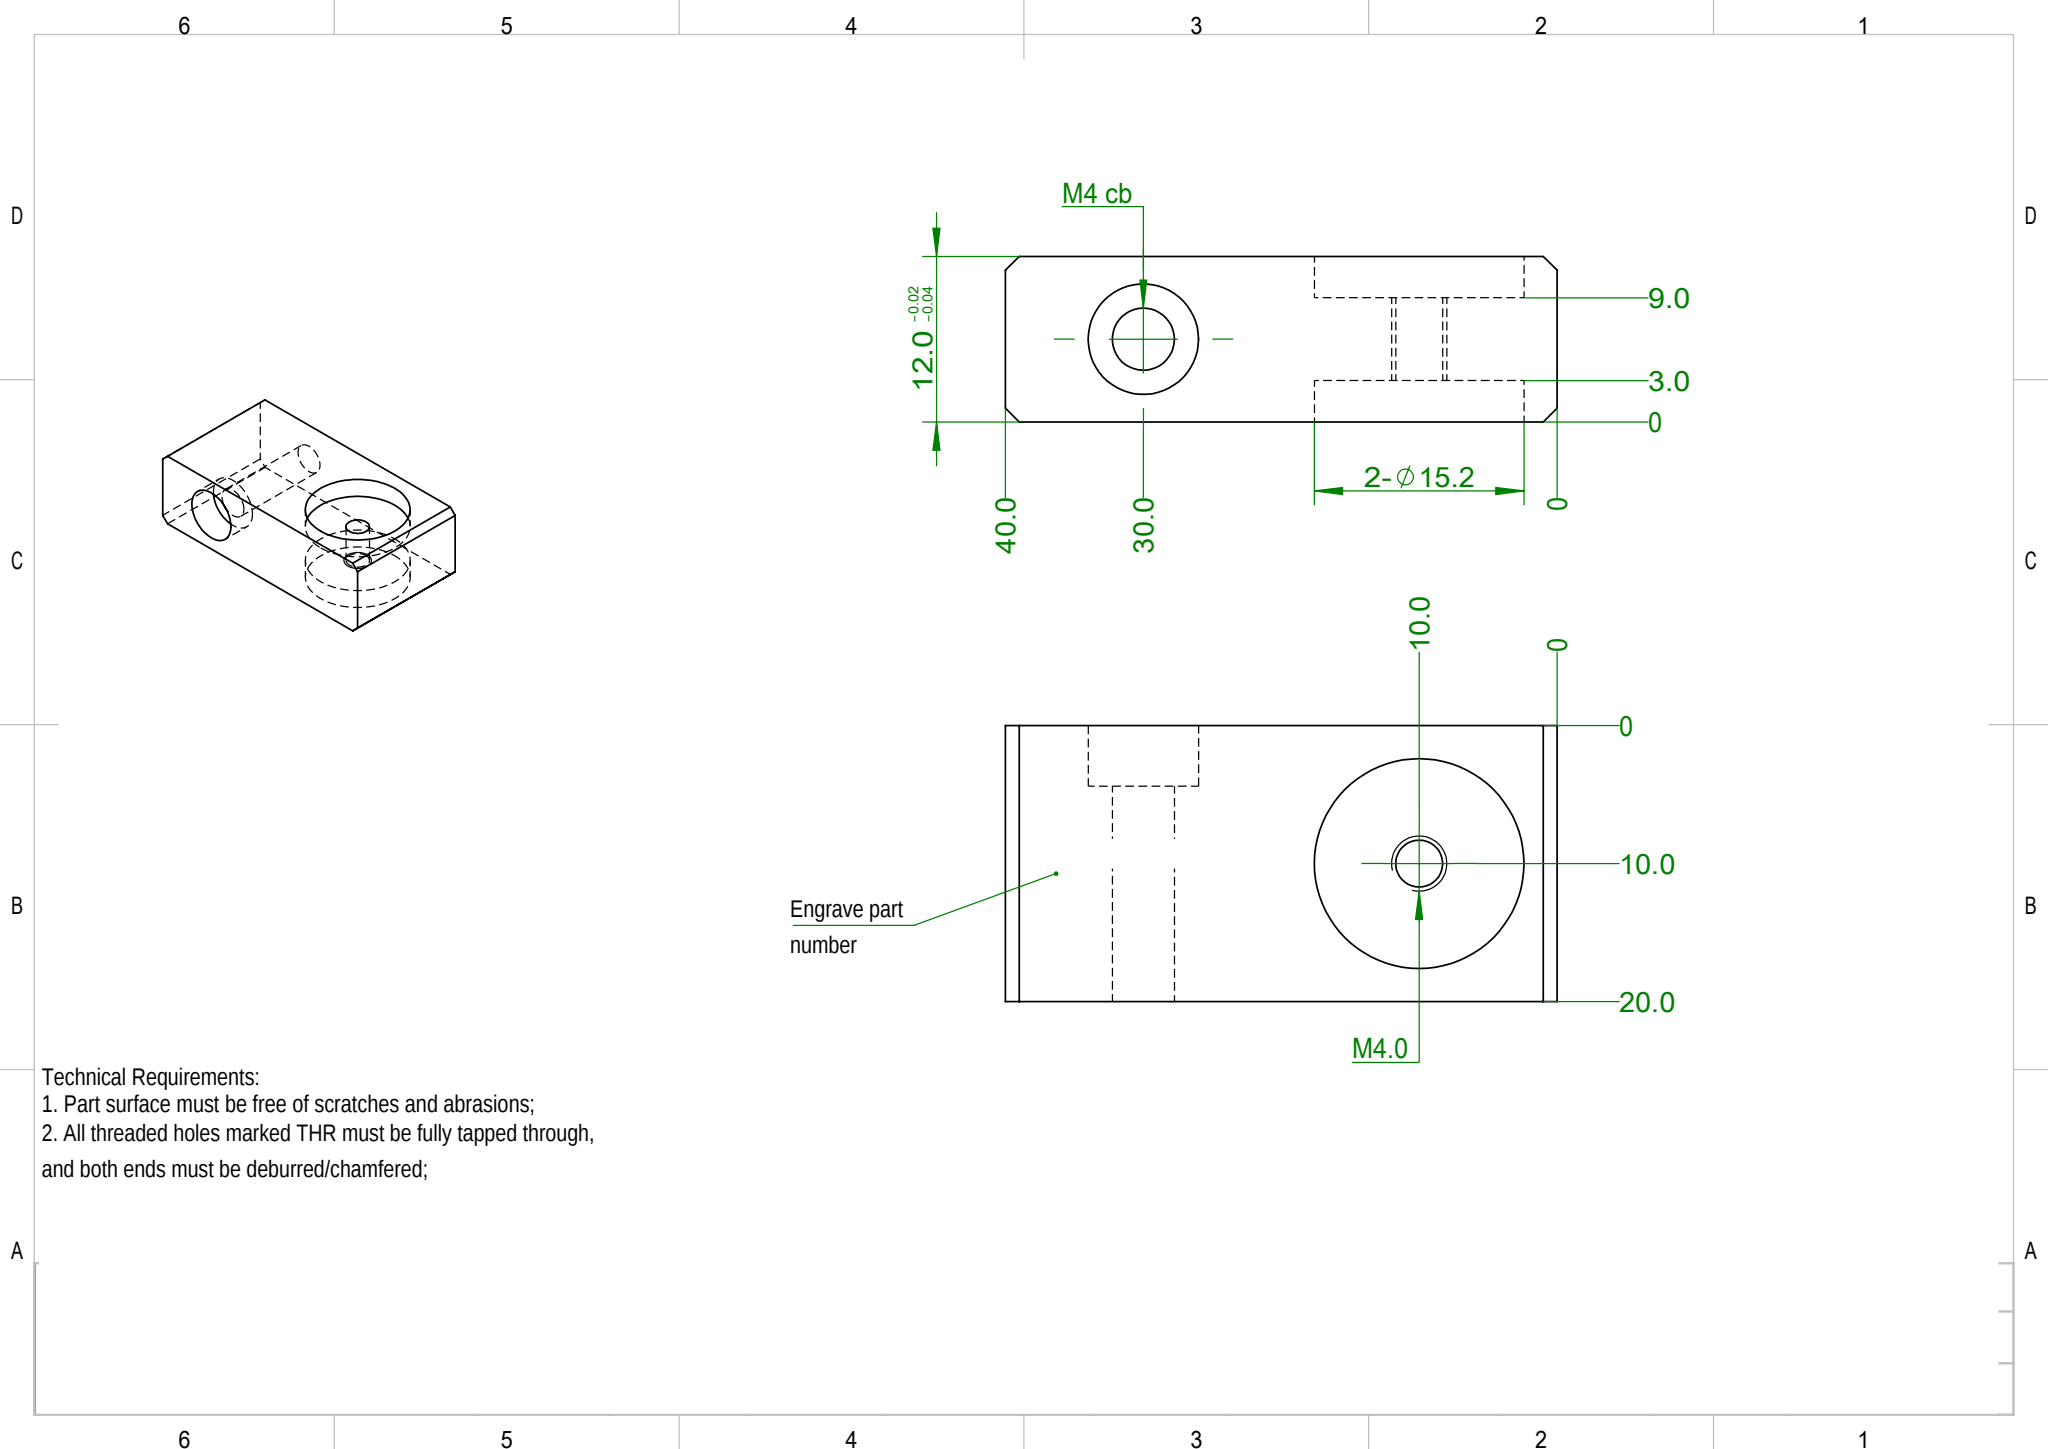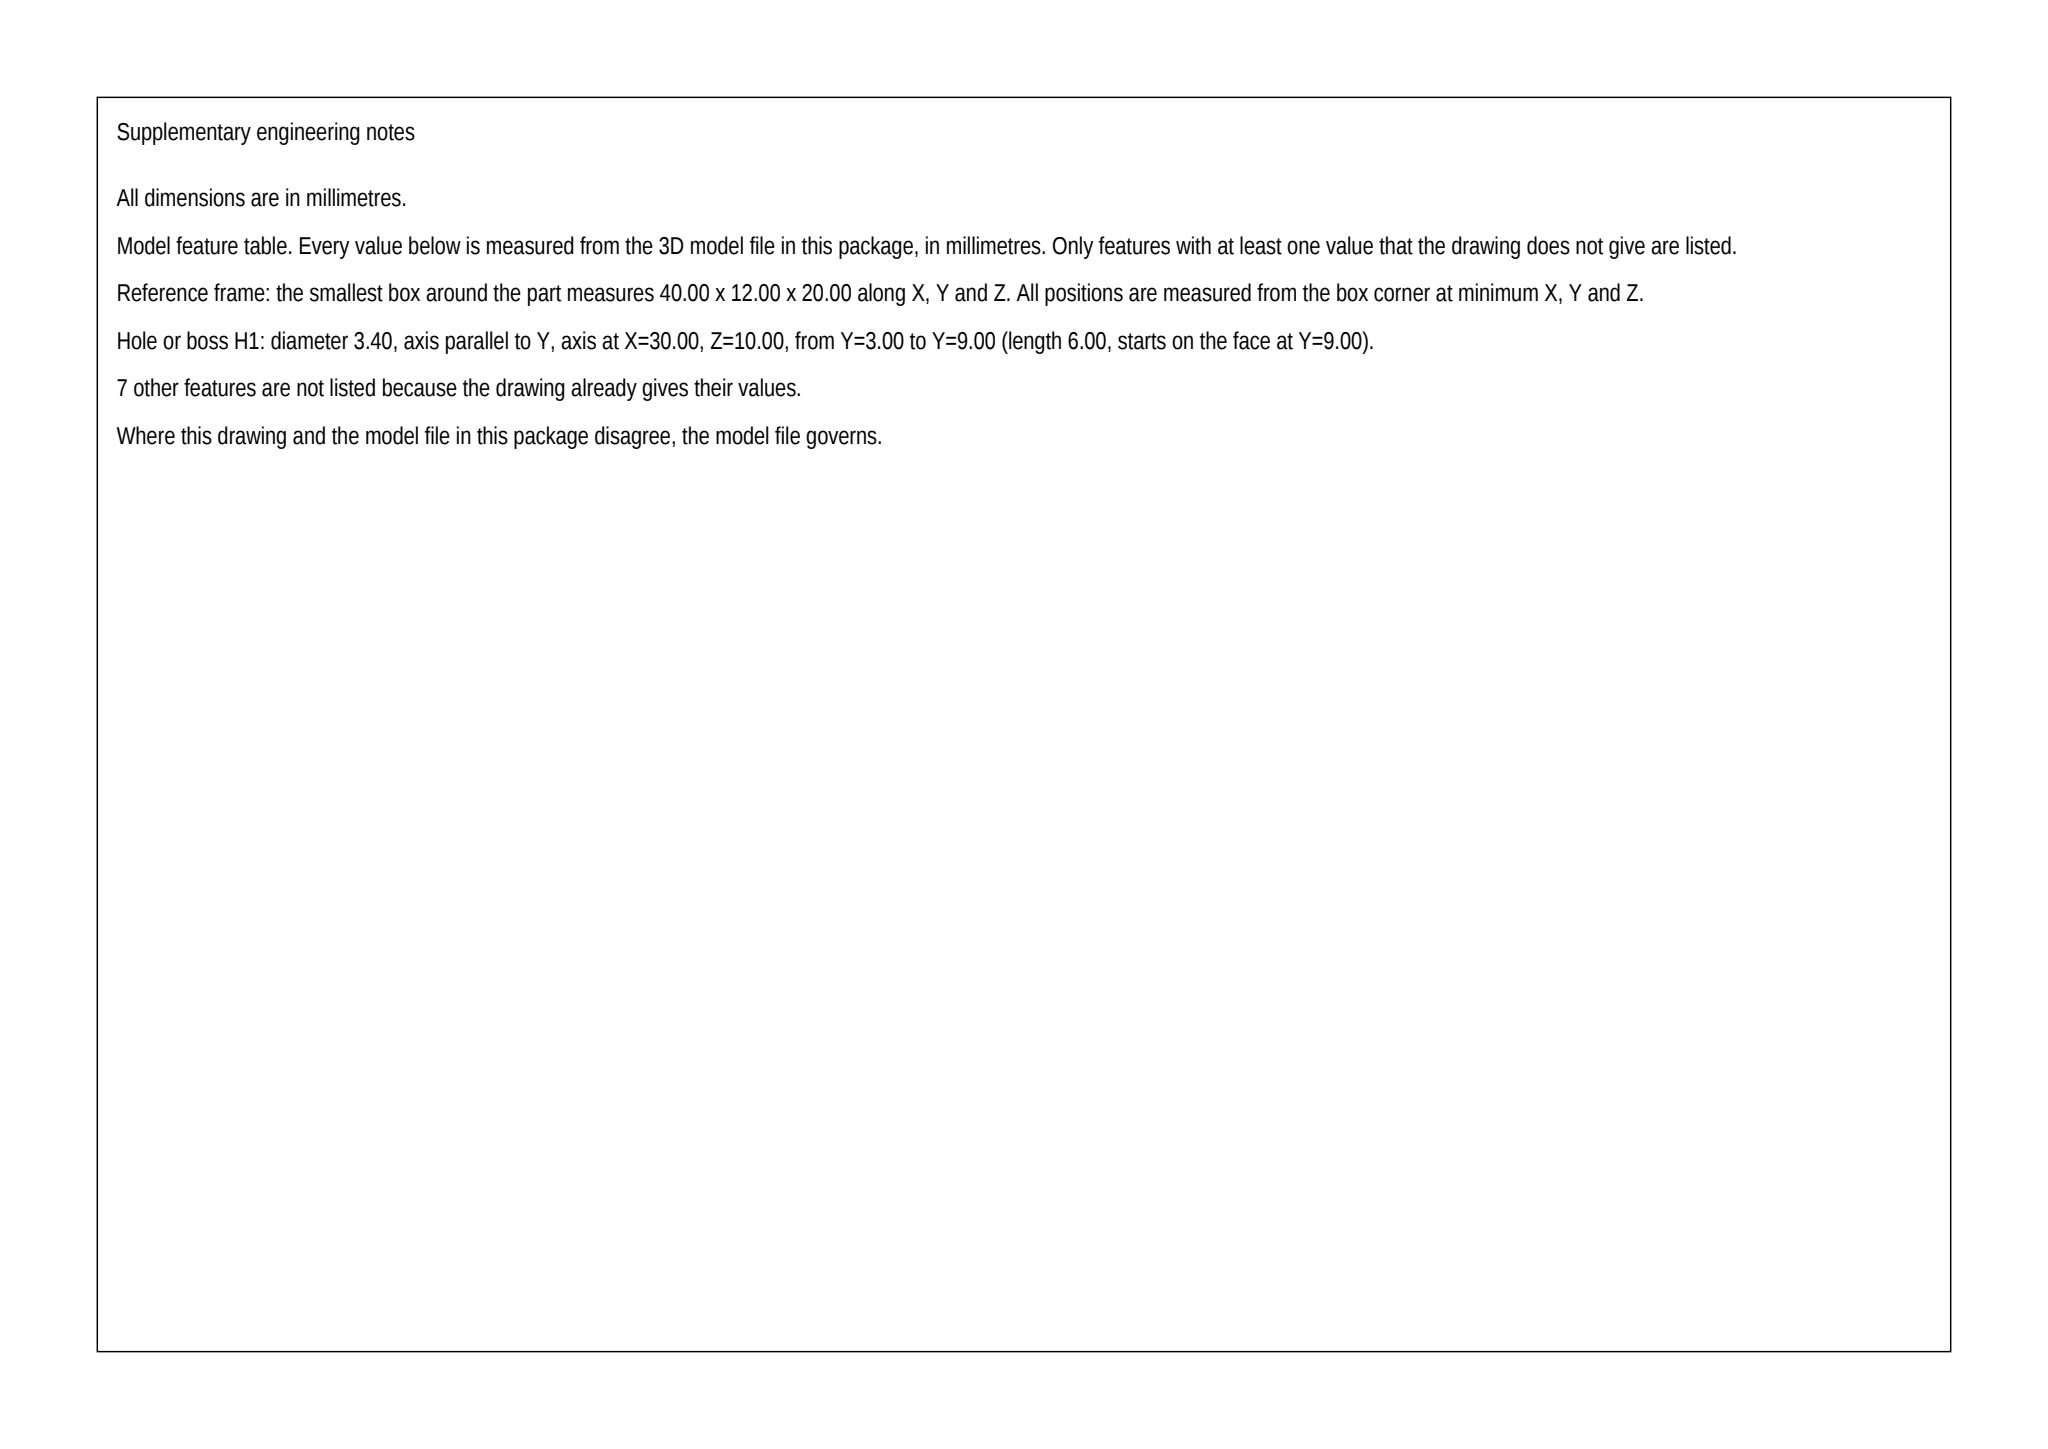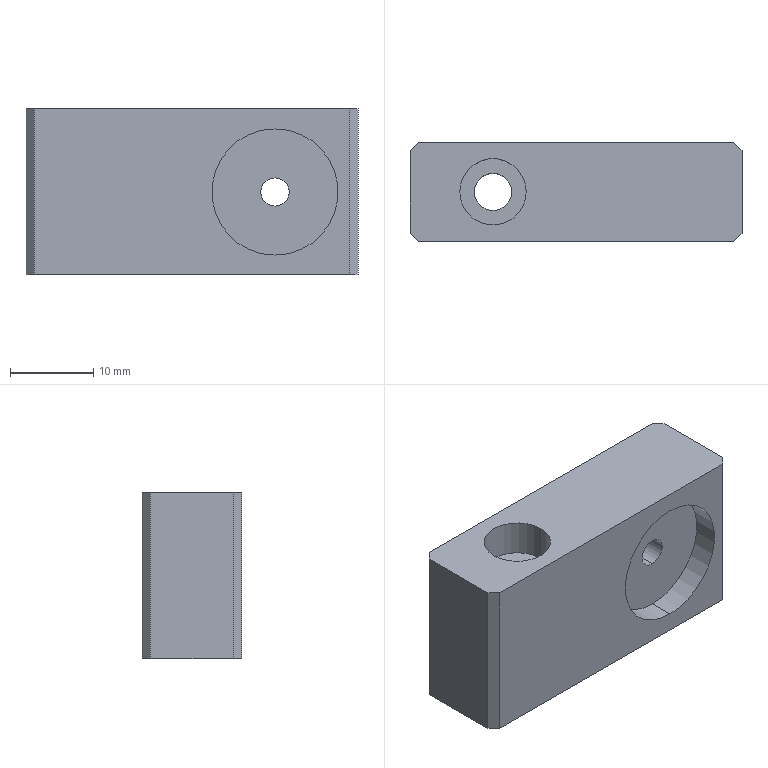Part | SolidWorks | mm | 1 solid | 23 faces | box 40 x 12 x 20 mm | volume 7947 mm3 | plane 13 | cylinder 10 | commonest cylinder face diameters 15.2 x4 8 x2 4.5 x2 3.4 x2
build123d program:
from build123d import *

# Parameters (mm, degrees)
SKETCH1_W                                       = 20
SKETCH1_H                                       = 12
BOSS_EXTRUDE1_DEPTH                             = 20
SKETCH4_R                                       = 7.6
CUT_EXTRUDE1_DEPTH                              = 3
SKETCH5_R                                       = 1.7
CUT_EXTRUDE2_DEPTH                              = 10
MOVE_FACE1_BY                                   = 20
M4_HEX_SOCKET_HEAD_CAP_SCREW_CBORE1_D           = 4.5
M4_HEX_SOCKET_HEAD_CAP_SCREW_CBORE1_CBORE_D     = 8
M4_HEX_SOCKET_HEAD_CAP_SCREW_CBORE1_CBORE_DEPTH = 4.4
CUT_EXTRUDE3_START                              = -3
SKETCH9_R                                       = 7.6
CUT_EXTRUDE3_DEPTH                              = 3
CHAMFER1_SIZE                                   = 1


with BuildPart() as part:
    # Sketch1 → Boss-Extrude1 (new body)
    with BuildSketch(Plane.XY):
        Rectangle(SKETCH1_W, SKETCH1_H)
    extrude(amount=BOSS_EXTRUDE1_DEPTH)

    # Sketch4 → Cut-Extrude1 (cut)
    with BuildSketch(Plane.XZ.offset(6)):
        with Locations(Location((0, 10, 0), (0, 0, 270))):
            Circle(SKETCH4_R)
    extrude(amount=-CUT_EXTRUDE1_DEPTH, mode=Mode.SUBTRACT)

    # Sketch5 → Cut-Extrude2 (cut)
    with BuildSketch(Plane.XZ.offset(3)):
        with Locations(Location((0, 10, 0), (0, 0, 270))):
            Circle(SKETCH5_R)
    extrude(amount=-CUT_EXTRUDE2_DEPTH, mode=Mode.SUBTRACT)

    # Move Face1: a face moved outward by 20.0
    extrude(part.faces().sort_by_distance((-10, 0, 10))[0], amount=MOVE_FACE1_BY, dir=(-1, 0, 0))

    # M4 Hex Socket Head Cap Screw CBORE1 (through all)
    with Locations(Plane.XY.offset(20)):
        with Locations((-20, 0)):
            CounterBoreHole(M4_HEX_SOCKET_HEAD_CAP_SCREW_CBORE1_D / 2, M4_HEX_SOCKET_HEAD_CAP_SCREW_CBORE1_CBORE_D / 2, M4_HEX_SOCKET_HEAD_CAP_SCREW_CBORE1_CBORE_DEPTH)

    # Sketch9 → Cut-Extrude3 (cut)
    with BuildSketch(Plane(origin=(0, 6, 0), x_dir=(1, 0, 0), z_dir=(0, 1, 0)).offset(CUT_EXTRUDE3_START)):
        with Locations(Location((0, -10, 0), (0, 0, 90))):
            Circle(SKETCH9_R)
    extrude(amount=CUT_EXTRUDE3_DEPTH, mode=Mode.SUBTRACT)

    # Chamfer1
    chamfer1_edges = [part.edges().sort_by_distance(p)[0] for p in [
        (10, -6, 10),
        (-30, -6, 10),
        (-30, 6, 10),
        (10, 6, 10),
    ]]
    chamfer(chamfer1_edges, length=CHAMFER1_SIZE)


solid = part.part
STEP:
#1=CARTESIAN_POINT('',(0.,3.,2.4));
#2=VERTEX_POINT('',#1);
#3=CARTESIAN_POINT('',(0.,3.,17.6));
#4=VERTEX_POINT('',#3);
#5=CARTESIAN_POINT('',(0.,3.,10.));
#6=DIRECTION('',(0.,1.,0.));
#7=DIRECTION('',(0.,0.,1.));
#8=AXIS2_PLACEMENT_3D('',#5,#6,#7);
#9=CIRCLE('',#8,7.6);
#10=EDGE_CURVE('',#2,#4,#9,.T.);
#11=ORIENTED_EDGE('',*,*,#10,.F.);
#12=CARTESIAN_POINT('',(0.,6.,2.4));
#13=VERTEX_POINT('',#12);
#14=CARTESIAN_POINT('',(0.,3.,2.4));
#15=DIRECTION('',(0.,1.,0.));
#16=VECTOR('',#15,1000.);
#17=LINE('',#14,#16);
#18=EDGE_CURVE('',#2,#13,#17,.T.);
#19=ORIENTED_EDGE('',*,*,#18,.T.);
#20=CARTESIAN_POINT('',(0.,6.,17.6));
#21=VERTEX_POINT('',#20);
#22=CARTESIAN_POINT('',(0.,6.,10.));
#23=DIRECTION('',(0.,1.,0.));
#24=DIRECTION('',(0.,0.,1.));
#25=AXIS2_PLACEMENT_3D('',#22,#23,#24);
#26=CIRCLE('',#25,7.6);
#27=EDGE_CURVE('',#13,#21,#26,.T.);
#28=ORIENTED_EDGE('',*,*,#27,.T.);
#29=CARTESIAN_POINT('',(0.,3.,17.6));
#30=DIRECTION('',(0.,1.,0.));
#31=VECTOR('',#30,1000.);
#32=LINE('',#29,#31);
#33=EDGE_CURVE('',#4,#21,#32,.T.);
#34=ORIENTED_EDGE('',*,*,#33,.F.);
#35=EDGE_LOOP('',(#11,#19,#28,#34));
#36=FACE_OUTER_BOUND('',#35,.T.);
#37=CARTESIAN_POINT('',(0.,3.,10.));
#38=DIRECTION('',(0.,1.,0.));
#39=DIRECTION('',(0.,0.,1.));
#40=AXIS2_PLACEMENT_3D('',#37,#38,#39);
#41=CYLINDRICAL_SURFACE('',#40,7.6);
#42=ADVANCED_FACE('',(#36),#41,.F.);
#43=CARTESIAN_POINT('',(-24.,-0.,15.6));
#44=VERTEX_POINT('',#43);
#45=CARTESIAN_POINT('',(-16.,-0.,15.6));
#46=VERTEX_POINT('',#45);
#47=CARTESIAN_POINT('',(-20.,-0.,15.6));
#48=DIRECTION('',(0.,0.,1.));
#49=DIRECTION('',(1.,0.,0.));
#50=AXIS2_PLACEMENT_3D('',#47,#48,#49);
#51=CIRCLE('',#50,4.);
#52=EDGE_CURVE('',#44,#46,#51,.T.);
#53=ORIENTED_EDGE('',*,*,#52,.F.);
#54=CARTESIAN_POINT('',(-24.,-0.,20.));
#55=VERTEX_POINT('',#54);
#56=CARTESIAN_POINT('',(-24.,-0.,20.));
#57=DIRECTION('',(0.,0.,1.));
#58=VECTOR('',#57,1000.);
#59=LINE('',#56,#58);
#60=EDGE_CURVE('',#44,#55,#59,.T.);
#61=ORIENTED_EDGE('',*,*,#60,.T.);
#62=CARTESIAN_POINT('',(-16.,-0.,20.));
#63=VERTEX_POINT('',#62);
#64=CARTESIAN_POINT('',(-20.,-0.,20.));
#65=DIRECTION('',(0.,0.,1.));
#66=DIRECTION('',(1.,0.,0.));
#67=AXIS2_PLACEMENT_3D('',#64,#65,#66);
#68=CIRCLE('',#67,4.);
#69=EDGE_CURVE('',#55,#63,#68,.T.);
#70=ORIENTED_EDGE('',*,*,#69,.T.);
#71=CARTESIAN_POINT('',(-16.,-0.,20.));
#72=DIRECTION('',(0.,0.,1.));
#73=VECTOR('',#72,1000.);
#74=LINE('',#71,#73);
#75=EDGE_CURVE('',#46,#63,#74,.T.);
#76=ORIENTED_EDGE('',*,*,#75,.F.);
#77=EDGE_LOOP('',(#53,#61,#70,#76));
#78=FACE_OUTER_BOUND('',#77,.T.);
#79=CARTESIAN_POINT('',(-20.,-0.,20.));
#80=DIRECTION('',(0.,0.,1.));
#81=DIRECTION('',(1.,0.,0.));
#82=AXIS2_PLACEMENT_3D('',#79,#80,#81);
#83=CYLINDRICAL_SURFACE('',#82,4.);
#84=ADVANCED_FACE('',(#78),#83,.F.);
#85=CARTESIAN_POINT('',(-22.25,-0.,0.));
#86=VERTEX_POINT('',#85);
#87=CARTESIAN_POINT('',(-17.75,-0.,0.));
#88=VERTEX_POINT('',#87);
#89=CARTESIAN_POINT('',(-20.,-0.,0.));
#90=DIRECTION('',(0.,0.,1.));
#91=DIRECTION('',(1.,0.,0.));
#92=AXIS2_PLACEMENT_3D('',#89,#90,#91);
#93=CIRCLE('',#92,2.25);
#94=EDGE_CURVE('',#86,#88,#93,.T.);
#95=ORIENTED_EDGE('',*,*,#94,.F.);
#96=CARTESIAN_POINT('',(-22.25,-0.,15.6));
#97=VERTEX_POINT('',#96);
#98=CARTESIAN_POINT('',(-22.25,-0.,20.));
#99=DIRECTION('',(0.,0.,1.));
#100=VECTOR('',#99,1000.);
#101=LINE('',#98,#100);
#102=EDGE_CURVE('',#86,#97,#101,.T.);
#103=ORIENTED_EDGE('',*,*,#102,.T.);
#104=CARTESIAN_POINT('',(-17.75,-0.,15.6));
#105=VERTEX_POINT('',#104);
#106=CARTESIAN_POINT('',(-20.,-0.,15.6));
#107=DIRECTION('',(0.,0.,1.));
#108=DIRECTION('',(1.,0.,0.));
#109=AXIS2_PLACEMENT_3D('',#106,#107,#108);
#110=CIRCLE('',#109,2.25);
#111=EDGE_CURVE('',#97,#105,#110,.T.);
#112=ORIENTED_EDGE('',*,*,#111,.T.);
#113=CARTESIAN_POINT('',(-17.75,-0.,20.));
#114=DIRECTION('',(0.,0.,1.));
#115=VECTOR('',#114,1000.);
#116=LINE('',#113,#115);
#117=EDGE_CURVE('',#88,#105,#116,.T.);
#118=ORIENTED_EDGE('',*,*,#117,.F.);
#119=EDGE_LOOP('',(#95,#103,#112,#118));
#120=FACE_OUTER_BOUND('',#119,.T.);
#121=CARTESIAN_POINT('',(-20.,-0.,20.));
#122=DIRECTION('',(0.,0.,1.));
#123=DIRECTION('',(1.,0.,0.));
#124=AXIS2_PLACEMENT_3D('',#121,#122,#123);
#125=CYLINDRICAL_SURFACE('',#124,2.25);
#126=ADVANCED_FACE('',(#120),#125,.F.);
#127=CARTESIAN_POINT('',(0.,-3.,17.6));
#128=VERTEX_POINT('',#127);
#129=CARTESIAN_POINT('',(0.,-3.,2.4));
#130=VERTEX_POINT('',#129);
#131=CARTESIAN_POINT('',(0.,-3.,10.));
#132=DIRECTION('',(0.,-1.,0.));
#133=DIRECTION('',(0.,0.,-1.));
#134=AXIS2_PLACEMENT_3D('',#131,#132,#133);
#135=CIRCLE('',#134,7.6);
#136=EDGE_CURVE('',#128,#130,#135,.T.);
#137=ORIENTED_EDGE('',*,*,#136,.F.);
#138=CARTESIAN_POINT('',(0.,-6.,17.6));
#139=VERTEX_POINT('',#138);
#140=CARTESIAN_POINT('',(0.,-3.,17.6));
#141=DIRECTION('',(0.,-1.,0.));
#142=VECTOR('',#141,1000.);
#143=LINE('',#140,#142);
#144=EDGE_CURVE('',#128,#139,#143,.T.);
#145=ORIENTED_EDGE('',*,*,#144,.T.);
#146=CARTESIAN_POINT('',(0.,-6.,2.4));
#147=VERTEX_POINT('',#146);
#148=CARTESIAN_POINT('',(0.,-6.,10.));
#149=DIRECTION('',(0.,-1.,0.));
#150=DIRECTION('',(0.,0.,-1.));
#151=AXIS2_PLACEMENT_3D('',#148,#149,#150);
#152=CIRCLE('',#151,7.6);
#153=EDGE_CURVE('',#139,#147,#152,.T.);
#154=ORIENTED_EDGE('',*,*,#153,.T.);
#155=CARTESIAN_POINT('',(0.,-3.,2.4));
#156=DIRECTION('',(0.,-1.,0.));
#157=VECTOR('',#156,1000.);
#158=LINE('',#155,#157);
#159=EDGE_CURVE('',#130,#147,#158,.T.);
#160=ORIENTED_EDGE('',*,*,#159,.F.);
#161=EDGE_LOOP('',(#137,#145,#154,#160));
#162=FACE_OUTER_BOUND('',#161,.T.);
#163=CARTESIAN_POINT('',(0.,-3.,10.));
#164=DIRECTION('',(0.,-1.,0.));
#165=DIRECTION('',(0.,0.,-1.));
#166=AXIS2_PLACEMENT_3D('',#163,#164,#165);
#167=CYLINDRICAL_SURFACE('',#166,7.6);
#168=ADVANCED_FACE('',(#162),#167,.F.);
#169=CARTESIAN_POINT('',(0.,3.,11.7));
#170=VERTEX_POINT('',#169);
#171=CARTESIAN_POINT('',(0.,3.,8.3));
#172=VERTEX_POINT('',#171);
#173=CARTESIAN_POINT('',(0.,3.,10.));
#174=DIRECTION('',(0.,-1.,0.));
#175=DIRECTION('',(0.,0.,1.));
#176=AXIS2_PLACEMENT_3D('',#173,#174,#175);
#177=CIRCLE('',#176,1.7);
#178=EDGE_CURVE('',#170,#172,#177,.T.);
#179=ORIENTED_EDGE('',*,*,#178,.F.);
#180=CARTESIAN_POINT('',(0.,-3.,11.7));
#181=VERTEX_POINT('',#180);
#182=CARTESIAN_POINT('',(0.,7.,11.7));
#183=DIRECTION('',(0.,-1.,0.));
#184=VECTOR('',#183,1000.);
#185=LINE('',#182,#184);
#186=EDGE_CURVE('',#170,#181,#185,.T.);
#187=ORIENTED_EDGE('',*,*,#186,.T.);
#188=CARTESIAN_POINT('',(0.,-3.,8.3));
#189=VERTEX_POINT('',#188);
#190=CARTESIAN_POINT('',(0.,-3.,10.));
#191=DIRECTION('',(0.,-1.,0.));
#192=DIRECTION('',(0.,0.,-1.));
#193=AXIS2_PLACEMENT_3D('',#190,#191,#192);
#194=CIRCLE('',#193,1.7);
#195=EDGE_CURVE('',#181,#189,#194,.T.);
#196=ORIENTED_EDGE('',*,*,#195,.T.);
#197=CARTESIAN_POINT('',(0.,7.,8.3));
#198=DIRECTION('',(0.,-1.,0.));
#199=VECTOR('',#198,1000.);
#200=LINE('',#197,#199);
#201=EDGE_CURVE('',#172,#189,#200,.T.);
#202=ORIENTED_EDGE('',*,*,#201,.F.);
#203=EDGE_LOOP('',(#179,#187,#196,#202));
#204=FACE_OUTER_BOUND('',#203,.T.);
#205=CARTESIAN_POINT('',(0.,7.,10.));
#206=DIRECTION('',(0.,-1.,0.));
#207=DIRECTION('',(0.,0.,-1.));
#208=AXIS2_PLACEMENT_3D('',#205,#206,#207);
#209=CYLINDRICAL_SURFACE('',#208,1.7);
#210=ADVANCED_FACE('',(#204),#209,.F.);
#211=ORIENTED_EDGE('',*,*,#186,.F.);
#212=CARTESIAN_POINT('',(0.,3.,10.));
#213=DIRECTION('',(0.,-1.,0.));
#214=DIRECTION('',(0.,0.,1.));
#215=AXIS2_PLACEMENT_3D('',#212,#213,#214);
#216=CIRCLE('',#215,1.7);
#217=EDGE_CURVE('',#172,#170,#216,.T.);
#218=ORIENTED_EDGE('',*,*,#217,.F.);
#219=ORIENTED_EDGE('',*,*,#201,.T.);
#220=CARTESIAN_POINT('',(0.,-3.,10.));
#221=DIRECTION('',(0.,-1.,0.));
#222=DIRECTION('',(0.,0.,-1.));
#223=AXIS2_PLACEMENT_3D('',#220,#221,#222);
#224=CIRCLE('',#223,1.7);
#225=EDGE_CURVE('',#189,#181,#224,.T.);
#226=ORIENTED_EDGE('',*,*,#225,.T.);
#227=EDGE_LOOP('',(#211,#218,#219,#226));
#228=FACE_OUTER_BOUND('',#227,.T.);
#229=CARTESIAN_POINT('',(0.,7.,10.));
#230=DIRECTION('',(0.,-1.,0.));
#231=DIRECTION('',(0.,0.,-1.));
#232=AXIS2_PLACEMENT_3D('',#229,#230,#231);
#233=CYLINDRICAL_SURFACE('',#232,1.7);
#234=ADVANCED_FACE('',(#228),#233,.F.);
#235=CARTESIAN_POINT('',(10.,-5.,20.));
#236=VERTEX_POINT('',#235);
#237=CARTESIAN_POINT('',(10.,5.,20.));
#238=VERTEX_POINT('',#237);
#239=CARTESIAN_POINT('',(10.,-6.,20.));
#240=DIRECTION('',(0.,1.,0.));
#241=VECTOR('',#240,1000.);
#242=LINE('',#239,#241);
#243=EDGE_CURVE('',#236,#238,#242,.T.);
#244=ORIENTED_EDGE('',*,*,#243,.F.);
#245=CARTESIAN_POINT('',(10.,-5.,0.));
#246=VERTEX_POINT('',#245);
#247=CARTESIAN_POINT('',(10.,-5.,20.));
#248=DIRECTION('',(0.,0.,-1.));
#249=VECTOR('',#248,1000.);
#250=LINE('',#247,#249);
#251=EDGE_CURVE('',#236,#246,#250,.T.);
#252=ORIENTED_EDGE('',*,*,#251,.T.);
#253=CARTESIAN_POINT('',(10.,5.,0.));
#254=VERTEX_POINT('',#253);
#255=CARTESIAN_POINT('',(10.,-6.,0.));
#256=DIRECTION('',(0.,1.,0.));
#257=VECTOR('',#256,1000.);
#258=LINE('',#255,#257);
#259=EDGE_CURVE('',#246,#254,#258,.T.);
#260=ORIENTED_EDGE('',*,*,#259,.T.);
#261=CARTESIAN_POINT('',(10.,5.,20.));
#262=DIRECTION('',(0.,0.,1.));
#263=VECTOR('',#262,1000.);
#264=LINE('',#261,#263);
#265=EDGE_CURVE('',#254,#238,#264,.T.);
#266=ORIENTED_EDGE('',*,*,#265,.T.);
#267=EDGE_LOOP('',(#244,#252,#260,#266));
#268=FACE_OUTER_BOUND('',#267,.T.);
#269=CARTESIAN_POINT('',(10.,-6.,20.));
#270=DIRECTION('',(-1.,0.,0.));
#271=DIRECTION('',(0.,0.,1.));
#272=AXIS2_PLACEMENT_3D('',#269,#270,#271);
#273=PLANE('',#272);
#274=ADVANCED_FACE('',(#268),#273,.F.);
#275=CARTESIAN_POINT('',(0.,6.,10.));
#276=DIRECTION('',(0.,1.,0.));
#277=DIRECTION('',(0.,0.,1.));
#278=AXIS2_PLACEMENT_3D('',#275,#276,#277);
#279=CIRCLE('',#278,7.6);
#280=EDGE_CURVE('',#21,#13,#279,.T.);
#281=ORIENTED_EDGE('',*,*,#280,.F.);
#282=ORIENTED_EDGE('',*,*,#27,.F.);
#283=EDGE_LOOP('',(#281,#282));
#284=FACE_BOUND('',#283,.T.);
#285=CARTESIAN_POINT('',(9.,6.,0.));
#286=VERTEX_POINT('',#285);
#287=CARTESIAN_POINT('',(-29.,6.,0.));
#288=VERTEX_POINT('',#287);
#289=CARTESIAN_POINT('',(-10.,6.,0.));
#290=DIRECTION('',(-1.,0.,0.));
#291=VECTOR('',#290,1000.);
#292=LINE('',#289,#291);
#293=EDGE_CURVE('',#286,#288,#292,.T.);
#294=ORIENTED_EDGE('',*,*,#293,.T.);
#295=CARTESIAN_POINT('',(-29.,6.,20.));
#296=VERTEX_POINT('',#295);
#297=CARTESIAN_POINT('',(-29.,6.,20.));
#298=DIRECTION('',(0.,0.,1.));
#299=VECTOR('',#298,1000.);
#300=LINE('',#297,#299);
#301=EDGE_CURVE('',#288,#296,#300,.T.);
#302=ORIENTED_EDGE('',*,*,#301,.T.);
#303=CARTESIAN_POINT('',(9.,6.,20.));
#304=VERTEX_POINT('',#303);
#305=CARTESIAN_POINT('',(-10.,6.,20.));
#306=DIRECTION('',(-1.,0.,0.));
#307=VECTOR('',#306,1000.);
#308=LINE('',#305,#307);
#309=EDGE_CURVE('',#304,#296,#308,.T.);
#310=ORIENTED_EDGE('',*,*,#309,.F.);
#311=CARTESIAN_POINT('',(9.,6.,20.));
#312=DIRECTION('',(0.,0.,-1.));
#313=VECTOR('',#312,1000.);
#314=LINE('',#311,#313);
#315=EDGE_CURVE('',#304,#286,#314,.T.);
#316=ORIENTED_EDGE('',*,*,#315,.T.);
#317=EDGE_LOOP('',(#294,#302,#310,#316));
#318=FACE_OUTER_BOUND('',#317,.T.);
#319=CARTESIAN_POINT('',(-10.,6.,20.));
#320=DIRECTION('',(0.,-1.,0.));
#321=DIRECTION('',(0.,0.,-1.));
#322=AXIS2_PLACEMENT_3D('',#319,#320,#321);
#323=PLANE('',#322);
#324=ADVANCED_FACE('',(#284,#318),#323,.F.);
#325=CARTESIAN_POINT('',(-30.,5.,0.));
#326=VERTEX_POINT('',#325);
#327=CARTESIAN_POINT('',(-30.,-5.,0.));
#328=VERTEX_POINT('',#327);
#329=CARTESIAN_POINT('',(-30.,0.,0.));
#330=DIRECTION('',(0.,-1.,0.));
#331=VECTOR('',#330,1000.);
#332=LINE('',#329,#331);
#333=EDGE_CURVE('',#326,#328,#332,.T.);
#334=ORIENTED_EDGE('',*,*,#333,.T.);
#335=CARTESIAN_POINT('',(-30.,-5.,20.));
#336=VERTEX_POINT('',#335);
#337=CARTESIAN_POINT('',(-30.,-5.,20.));
#338=DIRECTION('',(0.,0.,1.));
#339=VECTOR('',#338,1000.);
#340=LINE('',#337,#339);
#341=EDGE_CURVE('',#328,#336,#340,.T.);
#342=ORIENTED_EDGE('',*,*,#341,.T.);
#343=CARTESIAN_POINT('',(-30.,5.,20.));
#344=VERTEX_POINT('',#343);
#345=CARTESIAN_POINT('',(-30.,0.,20.));
#346=DIRECTION('',(0.,-1.,0.));
#347=VECTOR('',#346,1000.);
#348=LINE('',#345,#347);
#349=EDGE_CURVE('',#344,#336,#348,.T.);
#350=ORIENTED_EDGE('',*,*,#349,.F.);
#351=CARTESIAN_POINT('',(-30.,5.,20.));
#352=DIRECTION('',(0.,0.,-1.));
#353=VECTOR('',#352,1000.);
#354=LINE('',#351,#353);
#355=EDGE_CURVE('',#344,#326,#354,.T.);
#356=ORIENTED_EDGE('',*,*,#355,.T.);
#357=EDGE_LOOP('',(#334,#342,#350,#356));
#358=FACE_OUTER_BOUND('',#357,.T.);
#359=CARTESIAN_POINT('',(-30.,-6.,20.));
#360=DIRECTION('',(1.,0.,0.));
#361=DIRECTION('',(0.,0.,-1.));
#362=AXIS2_PLACEMENT_3D('',#359,#360,#361);
#363=PLANE('',#362);
#364=ADVANCED_FACE('',(#358),#363,.F.);
#365=CARTESIAN_POINT('',(0.,-6.,10.));
#366=DIRECTION('',(0.,-1.,0.));
#367=DIRECTION('',(0.,0.,-1.));
#368=AXIS2_PLACEMENT_3D('',#365,#366,#367);
#369=CIRCLE('',#368,7.6);
#370=EDGE_CURVE('',#147,#139,#369,.T.);
#371=ORIENTED_EDGE('',*,*,#370,.F.);
#372=ORIENTED_EDGE('',*,*,#153,.F.);
#373=EDGE_LOOP('',(#371,#372));
#374=FACE_BOUND('',#373,.T.);
#375=CARTESIAN_POINT('',(-29.,-6.,20.));
#376=VERTEX_POINT('',#375);
#377=CARTESIAN_POINT('',(9.,-6.,20.));
#378=VERTEX_POINT('',#377);
#379=CARTESIAN_POINT('',(-10.,-6.,20.));
#380=DIRECTION('',(1.,0.,0.));
#381=VECTOR('',#380,1000.);
#382=LINE('',#379,#381);
#383=EDGE_CURVE('',#376,#378,#382,.T.);
#384=ORIENTED_EDGE('',*,*,#383,.F.);
#385=CARTESIAN_POINT('',(-29.,-6.,0.));
#386=VERTEX_POINT('',#385);
#387=CARTESIAN_POINT('',(-29.,-6.,20.));
#388=DIRECTION('',(0.,0.,-1.));
#389=VECTOR('',#388,1000.);
#390=LINE('',#387,#389);
#391=EDGE_CURVE('',#376,#386,#390,.T.);
#392=ORIENTED_EDGE('',*,*,#391,.T.);
#393=CARTESIAN_POINT('',(9.,-6.,0.));
#394=VERTEX_POINT('',#393);
#395=CARTESIAN_POINT('',(-10.,-6.,0.));
#396=DIRECTION('',(1.,0.,0.));
#397=VECTOR('',#396,1000.);
#398=LINE('',#395,#397);
#399=EDGE_CURVE('',#386,#394,#398,.T.);
#400=ORIENTED_EDGE('',*,*,#399,.T.);
#401=CARTESIAN_POINT('',(9.,-6.,20.));
#402=DIRECTION('',(0.,0.,1.));
#403=VECTOR('',#402,1000.);
#404=LINE('',#401,#403);
#405=EDGE_CURVE('',#394,#378,#404,.T.);
#406=ORIENTED_EDGE('',*,*,#405,.T.);
#407=EDGE_LOOP('',(#384,#392,#400,#406));
#408=FACE_OUTER_BOUND('',#407,.T.);
#409=CARTESIAN_POINT('',(-10.,-6.,20.));
#410=DIRECTION('',(0.,1.,0.));
#411=DIRECTION('',(0.,0.,1.));
#412=AXIS2_PLACEMENT_3D('',#409,#410,#411);
#413=PLANE('',#412);
#414=ADVANCED_FACE('',(#374,#408),#413,.F.);
#415=CARTESIAN_POINT('',(-20.,-0.,20.));
#416=DIRECTION('',(0.,0.,1.));
#417=DIRECTION('',(1.,0.,0.));
#418=AXIS2_PLACEMENT_3D('',#415,#416,#417);
#419=CIRCLE('',#418,4.);
#420=EDGE_CURVE('',#63,#55,#419,.T.);
#421=ORIENTED_EDGE('',*,*,#420,.F.);
#422=ORIENTED_EDGE('',*,*,#69,.F.);
#423=EDGE_LOOP('',(#421,#422));
#424=FACE_BOUND('',#423,.T.);
#425=ORIENTED_EDGE('',*,*,#349,.T.);
#426=CARTESIAN_POINT('',(-29.,-6.,20.));
#427=DIRECTION('',(0.7071,-0.7071,0.));
#428=VECTOR('',#427,1000.);
#429=LINE('',#426,#428);
#430=EDGE_CURVE('',#336,#376,#429,.T.);
#431=ORIENTED_EDGE('',*,*,#430,.T.);
#432=ORIENTED_EDGE('',*,*,#383,.T.);
#433=CARTESIAN_POINT('',(10.,-5.,20.));
#434=DIRECTION('',(0.7071,0.7071,0.));
#435=VECTOR('',#434,1000.);
#436=LINE('',#433,#435);
#437=EDGE_CURVE('',#378,#236,#436,.T.);
#438=ORIENTED_EDGE('',*,*,#437,.T.);
#439=ORIENTED_EDGE('',*,*,#243,.T.);
#440=CARTESIAN_POINT('',(9.,6.,20.));
#441=DIRECTION('',(-0.7071,0.7071,0.));
#442=VECTOR('',#441,1000.);
#443=LINE('',#440,#442);
#444=EDGE_CURVE('',#238,#304,#443,.T.);
#445=ORIENTED_EDGE('',*,*,#444,.T.);
#446=ORIENTED_EDGE('',*,*,#309,.T.);
#447=CARTESIAN_POINT('',(-30.,5.,20.));
#448=DIRECTION('',(-0.7071,-0.7071,0.));
#449=VECTOR('',#448,1000.);
#450=LINE('',#447,#449);
#451=EDGE_CURVE('',#296,#344,#450,.T.);
#452=ORIENTED_EDGE('',*,*,#451,.T.);
#453=EDGE_LOOP('',(#425,#431,#432,#438,#439,#445,#446,#452));
#454=FACE_OUTER_BOUND('',#453,.T.);
#455=CARTESIAN_POINT('',(0.,0.,20.));
#456=DIRECTION('',(0.,0.,-1.));
#457=DIRECTION('',(-1.,0.,0.));
#458=AXIS2_PLACEMENT_3D('',#455,#456,#457);
#459=PLANE('',#458);
#460=ADVANCED_FACE('',(#424,#454),#459,.F.);
#461=CARTESIAN_POINT('',(-20.,-0.,0.));
#462=DIRECTION('',(0.,0.,1.));
#463=DIRECTION('',(1.,0.,0.));
#464=AXIS2_PLACEMENT_3D('',#461,#462,#463);
#465=CIRCLE('',#464,2.25);
#466=EDGE_CURVE('',#88,#86,#465,.T.);
#467=ORIENTED_EDGE('',*,*,#466,.T.);
#468=ORIENTED_EDGE('',*,*,#94,.T.);
#469=EDGE_LOOP('',(#467,#468));
#470=FACE_BOUND('',#469,.T.);
#471=ORIENTED_EDGE('',*,*,#399,.F.);
#472=CARTESIAN_POINT('',(-17.5,-17.5,0.));
#473=DIRECTION('',(-0.7071,0.7071,0.));
#474=VECTOR('',#473,1000.);
#475=LINE('',#472,#474);
#476=EDGE_CURVE('',#386,#328,#475,.T.);
#477=ORIENTED_EDGE('',*,*,#476,.T.);
#478=ORIENTED_EDGE('',*,*,#333,.F.);
#479=CARTESIAN_POINT('',(-17.5,17.5,0.));
#480=DIRECTION('',(0.7071,0.7071,0.));
#481=VECTOR('',#480,1000.);
#482=LINE('',#479,#481);
#483=EDGE_CURVE('',#326,#288,#482,.T.);
#484=ORIENTED_EDGE('',*,*,#483,.T.);
#485=ORIENTED_EDGE('',*,*,#293,.F.);
#486=CARTESIAN_POINT('',(7.5,7.5,0.));
#487=DIRECTION('',(0.7071,-0.7071,0.));
#488=VECTOR('',#487,1000.);
#489=LINE('',#486,#488);
#490=EDGE_CURVE('',#286,#254,#489,.T.);
#491=ORIENTED_EDGE('',*,*,#490,.T.);
#492=ORIENTED_EDGE('',*,*,#259,.F.);
#493=CARTESIAN_POINT('',(7.5,-7.5,0.));
#494=DIRECTION('',(-0.7071,-0.7071,0.));
#495=VECTOR('',#494,1000.);
#496=LINE('',#493,#495);
#497=EDGE_CURVE('',#246,#394,#496,.T.);
#498=ORIENTED_EDGE('',*,*,#497,.T.);
#499=EDGE_LOOP('',(#471,#477,#478,#484,#485,#491,#492,#498));
#500=FACE_OUTER_BOUND('',#499,.T.);
#501=CARTESIAN_POINT('',(0.,0.,0.));
#502=DIRECTION('',(0.,0.,-1.));
#503=DIRECTION('',(-1.,0.,0.));
#504=AXIS2_PLACEMENT_3D('',#501,#502,#503);
#505=PLANE('',#504);
#506=ADVANCED_FACE('',(#470,#500),#505,.T.);
#507=ORIENTED_EDGE('',*,*,#144,.F.);
#508=CARTESIAN_POINT('',(0.,-3.,10.));
#509=DIRECTION('',(0.,-1.,0.));
#510=DIRECTION('',(0.,0.,-1.));
#511=AXIS2_PLACEMENT_3D('',#508,#509,#510);
#512=CIRCLE('',#511,7.6);
#513=EDGE_CURVE('',#130,#128,#512,.T.);
#514=ORIENTED_EDGE('',*,*,#513,.F.);
#515=ORIENTED_EDGE('',*,*,#159,.T.);
#516=ORIENTED_EDGE('',*,*,#370,.T.);
#517=EDGE_LOOP('',(#507,#514,#515,#516));
#518=FACE_OUTER_BOUND('',#517,.T.);
#519=CARTESIAN_POINT('',(0.,-3.,10.));
#520=DIRECTION('',(0.,-1.,0.));
#521=DIRECTION('',(0.,0.,-1.));
#522=AXIS2_PLACEMENT_3D('',#519,#520,#521);
#523=CYLINDRICAL_SURFACE('',#522,7.6);
#524=ADVANCED_FACE('',(#518),#523,.F.);
#525=ORIENTED_EDGE('',*,*,#225,.F.);
#526=ORIENTED_EDGE('',*,*,#195,.F.);
#527=EDGE_LOOP('',(#525,#526));
#528=FACE_BOUND('',#527,.T.);
#529=ORIENTED_EDGE('',*,*,#513,.T.);
#530=ORIENTED_EDGE('',*,*,#136,.T.);
#531=EDGE_LOOP('',(#529,#530));
#532=FACE_OUTER_BOUND('',#531,.T.);
#533=CARTESIAN_POINT('',(0.,-3.,10.));
#534=DIRECTION('',(0.,-1.,0.));
#535=DIRECTION('',(0.,0.,-1.));
#536=AXIS2_PLACEMENT_3D('',#533,#534,#535);
#537=PLANE('',#536);
#538=ADVANCED_FACE('',(#528,#532),#537,.T.);
#539=ORIENTED_EDGE('',*,*,#102,.F.);
#540=ORIENTED_EDGE('',*,*,#466,.F.);
#541=ORIENTED_EDGE('',*,*,#117,.T.);
#542=CARTESIAN_POINT('',(-20.,-0.,15.6));
#543=DIRECTION('',(0.,0.,1.));
#544=DIRECTION('',(1.,0.,0.));
#545=AXIS2_PLACEMENT_3D('',#542,#543,#544);
#546=CIRCLE('',#545,2.25);
#547=EDGE_CURVE('',#105,#97,#546,.T.);
#548=ORIENTED_EDGE('',*,*,#547,.T.);
#549=EDGE_LOOP('',(#539,#540,#541,#548));
#550=FACE_OUTER_BOUND('',#549,.T.);
#551=CARTESIAN_POINT('',(-20.,-0.,20.));
#552=DIRECTION('',(0.,0.,1.));
#553=DIRECTION('',(1.,0.,0.));
#554=AXIS2_PLACEMENT_3D('',#551,#552,#553);
#555=CYLINDRICAL_SURFACE('',#554,2.25);
#556=ADVANCED_FACE('',(#550),#555,.F.);
#557=ORIENTED_EDGE('',*,*,#547,.F.);
#558=ORIENTED_EDGE('',*,*,#111,.F.);
#559=EDGE_LOOP('',(#557,#558));
#560=FACE_BOUND('',#559,.T.);
#561=CARTESIAN_POINT('',(-20.,-0.,15.6));
#562=DIRECTION('',(0.,0.,1.));
#563=DIRECTION('',(1.,0.,0.));
#564=AXIS2_PLACEMENT_3D('',#561,#562,#563);
#565=CIRCLE('',#564,4.);
#566=EDGE_CURVE('',#46,#44,#565,.T.);
#567=ORIENTED_EDGE('',*,*,#566,.T.);
#568=ORIENTED_EDGE('',*,*,#52,.T.);
#569=EDGE_LOOP('',(#567,#568));
#570=FACE_OUTER_BOUND('',#569,.T.);
#571=CARTESIAN_POINT('',(-17.75,-0.,15.6));
#572=DIRECTION('',(0.,0.,-1.));
#573=DIRECTION('',(-1.,0.,0.));
#574=AXIS2_PLACEMENT_3D('',#571,#572,#573);
#575=PLANE('',#574);
#576=ADVANCED_FACE('',(#560,#570),#575,.F.);
#577=ORIENTED_EDGE('',*,*,#60,.F.);
#578=ORIENTED_EDGE('',*,*,#566,.F.);
#579=ORIENTED_EDGE('',*,*,#75,.T.);
#580=ORIENTED_EDGE('',*,*,#420,.T.);
#581=EDGE_LOOP('',(#577,#578,#579,#580));
#582=FACE_OUTER_BOUND('',#581,.T.);
#583=CARTESIAN_POINT('',(-20.,-0.,20.));
#584=DIRECTION('',(0.,0.,1.));
#585=DIRECTION('',(1.,0.,0.));
#586=AXIS2_PLACEMENT_3D('',#583,#584,#585);
#587=CYLINDRICAL_SURFACE('',#586,4.);
#588=ADVANCED_FACE('',(#582),#587,.F.);
#589=CARTESIAN_POINT('',(0.,3.,10.));
#590=DIRECTION('',(0.,1.,0.));
#591=DIRECTION('',(0.,0.,1.));
#592=AXIS2_PLACEMENT_3D('',#589,#590,#591);
#593=CIRCLE('',#592,7.6);
#594=EDGE_CURVE('',#4,#2,#593,.T.);
#595=ORIENTED_EDGE('',*,*,#594,.T.);
#596=ORIENTED_EDGE('',*,*,#10,.T.);
#597=EDGE_LOOP('',(#595,#596));
#598=FACE_OUTER_BOUND('',#597,.T.);
#599=ORIENTED_EDGE('',*,*,#217,.T.);
#600=ORIENTED_EDGE('',*,*,#178,.T.);
#601=EDGE_LOOP('',(#599,#600));
#602=FACE_BOUND('',#601,.T.);
#603=CARTESIAN_POINT('',(0.,3.,10.));
#604=DIRECTION('',(0.,1.,0.));
#605=DIRECTION('',(0.,0.,1.));
#606=AXIS2_PLACEMENT_3D('',#603,#604,#605);
#607=PLANE('',#606);
#608=ADVANCED_FACE('',(#598,#602),#607,.T.);
#609=ORIENTED_EDGE('',*,*,#18,.F.);
#610=ORIENTED_EDGE('',*,*,#594,.F.);
#611=ORIENTED_EDGE('',*,*,#33,.T.);
#612=ORIENTED_EDGE('',*,*,#280,.T.);
#613=EDGE_LOOP('',(#609,#610,#611,#612));
#614=FACE_OUTER_BOUND('',#613,.T.);
#615=CARTESIAN_POINT('',(0.,3.,10.));
#616=DIRECTION('',(0.,1.,0.));
#617=DIRECTION('',(0.,0.,1.));
#618=AXIS2_PLACEMENT_3D('',#615,#616,#617);
#619=CYLINDRICAL_SURFACE('',#618,7.6);
#620=ADVANCED_FACE('',(#614),#619,.F.);
#621=ORIENTED_EDGE('',*,*,#430,.F.);
#622=ORIENTED_EDGE('',*,*,#341,.F.);
#623=ORIENTED_EDGE('',*,*,#476,.F.);
#624=ORIENTED_EDGE('',*,*,#391,.F.);
#625=EDGE_LOOP('',(#621,#622,#623,#624));
#626=FACE_OUTER_BOUND('',#625,.T.);
#627=CARTESIAN_POINT('',(-29.,-6.,20.));
#628=DIRECTION('',(0.7071,0.7071,0.));
#629=DIRECTION('',(0.,0.,-1.));
#630=AXIS2_PLACEMENT_3D('',#627,#628,#629);
#631=PLANE('',#630);
#632=ADVANCED_FACE('',(#626),#631,.F.);
#633=ORIENTED_EDGE('',*,*,#451,.F.);
#634=ORIENTED_EDGE('',*,*,#301,.F.);
#635=ORIENTED_EDGE('',*,*,#483,.F.);
#636=ORIENTED_EDGE('',*,*,#355,.F.);
#637=EDGE_LOOP('',(#633,#634,#635,#636));
#638=FACE_OUTER_BOUND('',#637,.T.);
#639=CARTESIAN_POINT('',(-30.,5.,20.));
#640=DIRECTION('',(0.7071,-0.7071,0.));
#641=DIRECTION('',(0.,0.,-1.));
#642=AXIS2_PLACEMENT_3D('',#639,#640,#641);
#643=PLANE('',#642);
#644=ADVANCED_FACE('',(#638),#643,.F.);
#645=ORIENTED_EDGE('',*,*,#437,.F.);
#646=ORIENTED_EDGE('',*,*,#405,.F.);
#647=ORIENTED_EDGE('',*,*,#497,.F.);
#648=ORIENTED_EDGE('',*,*,#251,.F.);
#649=EDGE_LOOP('',(#645,#646,#647,#648));
#650=FACE_OUTER_BOUND('',#649,.T.);
#651=CARTESIAN_POINT('',(10.,-5.,20.));
#652=DIRECTION('',(-0.7071,0.7071,0.));
#653=DIRECTION('',(0.,0.,-1.));
#654=AXIS2_PLACEMENT_3D('',#651,#652,#653);
#655=PLANE('',#654);
#656=ADVANCED_FACE('',(#650),#655,.F.);
#657=ORIENTED_EDGE('',*,*,#444,.F.);
#658=ORIENTED_EDGE('',*,*,#265,.F.);
#659=ORIENTED_EDGE('',*,*,#490,.F.);
#660=ORIENTED_EDGE('',*,*,#315,.F.);
#661=EDGE_LOOP('',(#657,#658,#659,#660));
#662=FACE_OUTER_BOUND('',#661,.T.);
#663=CARTESIAN_POINT('',(9.,6.,20.));
#664=DIRECTION('',(-0.7071,-0.7071,0.));
#665=DIRECTION('',(0.,0.,-1.));
#666=AXIS2_PLACEMENT_3D('',#663,#664,#665);
#667=PLANE('',#666);
#668=ADVANCED_FACE('',(#662),#667,.F.);
#669=CLOSED_SHELL('',(#42,#84,#126,#168,#210,#234,#274,#324,#364,#414,#460,#506,#524,#538,#556,#576,#588,#608,#620,#632,#644,#656,#668));
#670=MANIFOLD_SOLID_BREP('',#669);
#671=CARTESIAN_POINT('',(0.,0.,0.));
#672=DIRECTION('',(0.,0.,1.));
#673=DIRECTION('',(1.,0.,0.));
#674=AXIS2_PLACEMENT_3D('',#671,#672,#673);
#675=(LENGTH_UNIT()NAMED_UNIT(*)SI_UNIT(.MILLI.,.METRE.));
#676=UNCERTAINTY_MEASURE_WITH_UNIT(LENGTH_MEASURE(0.00001),#675,'','');
#677=(NAMED_UNIT(*)PLANE_ANGLE_UNIT()SI_UNIT($,.RADIAN.));
#678=(NAMED_UNIT(*)SI_UNIT($,.STERADIAN.)SOLID_ANGLE_UNIT());
#679=(GEOMETRIC_REPRESENTATION_CONTEXT(3)GLOBAL_UNCERTAINTY_ASSIGNED_CONTEXT((#676))GLOBAL_UNIT_ASSIGNED_CONTEXT((#675,#677,#678))REPRESENTATION_CONTEXT('',''));
#680=ADVANCED_BREP_SHAPE_REPRESENTATION('',(#670,#674),#679);